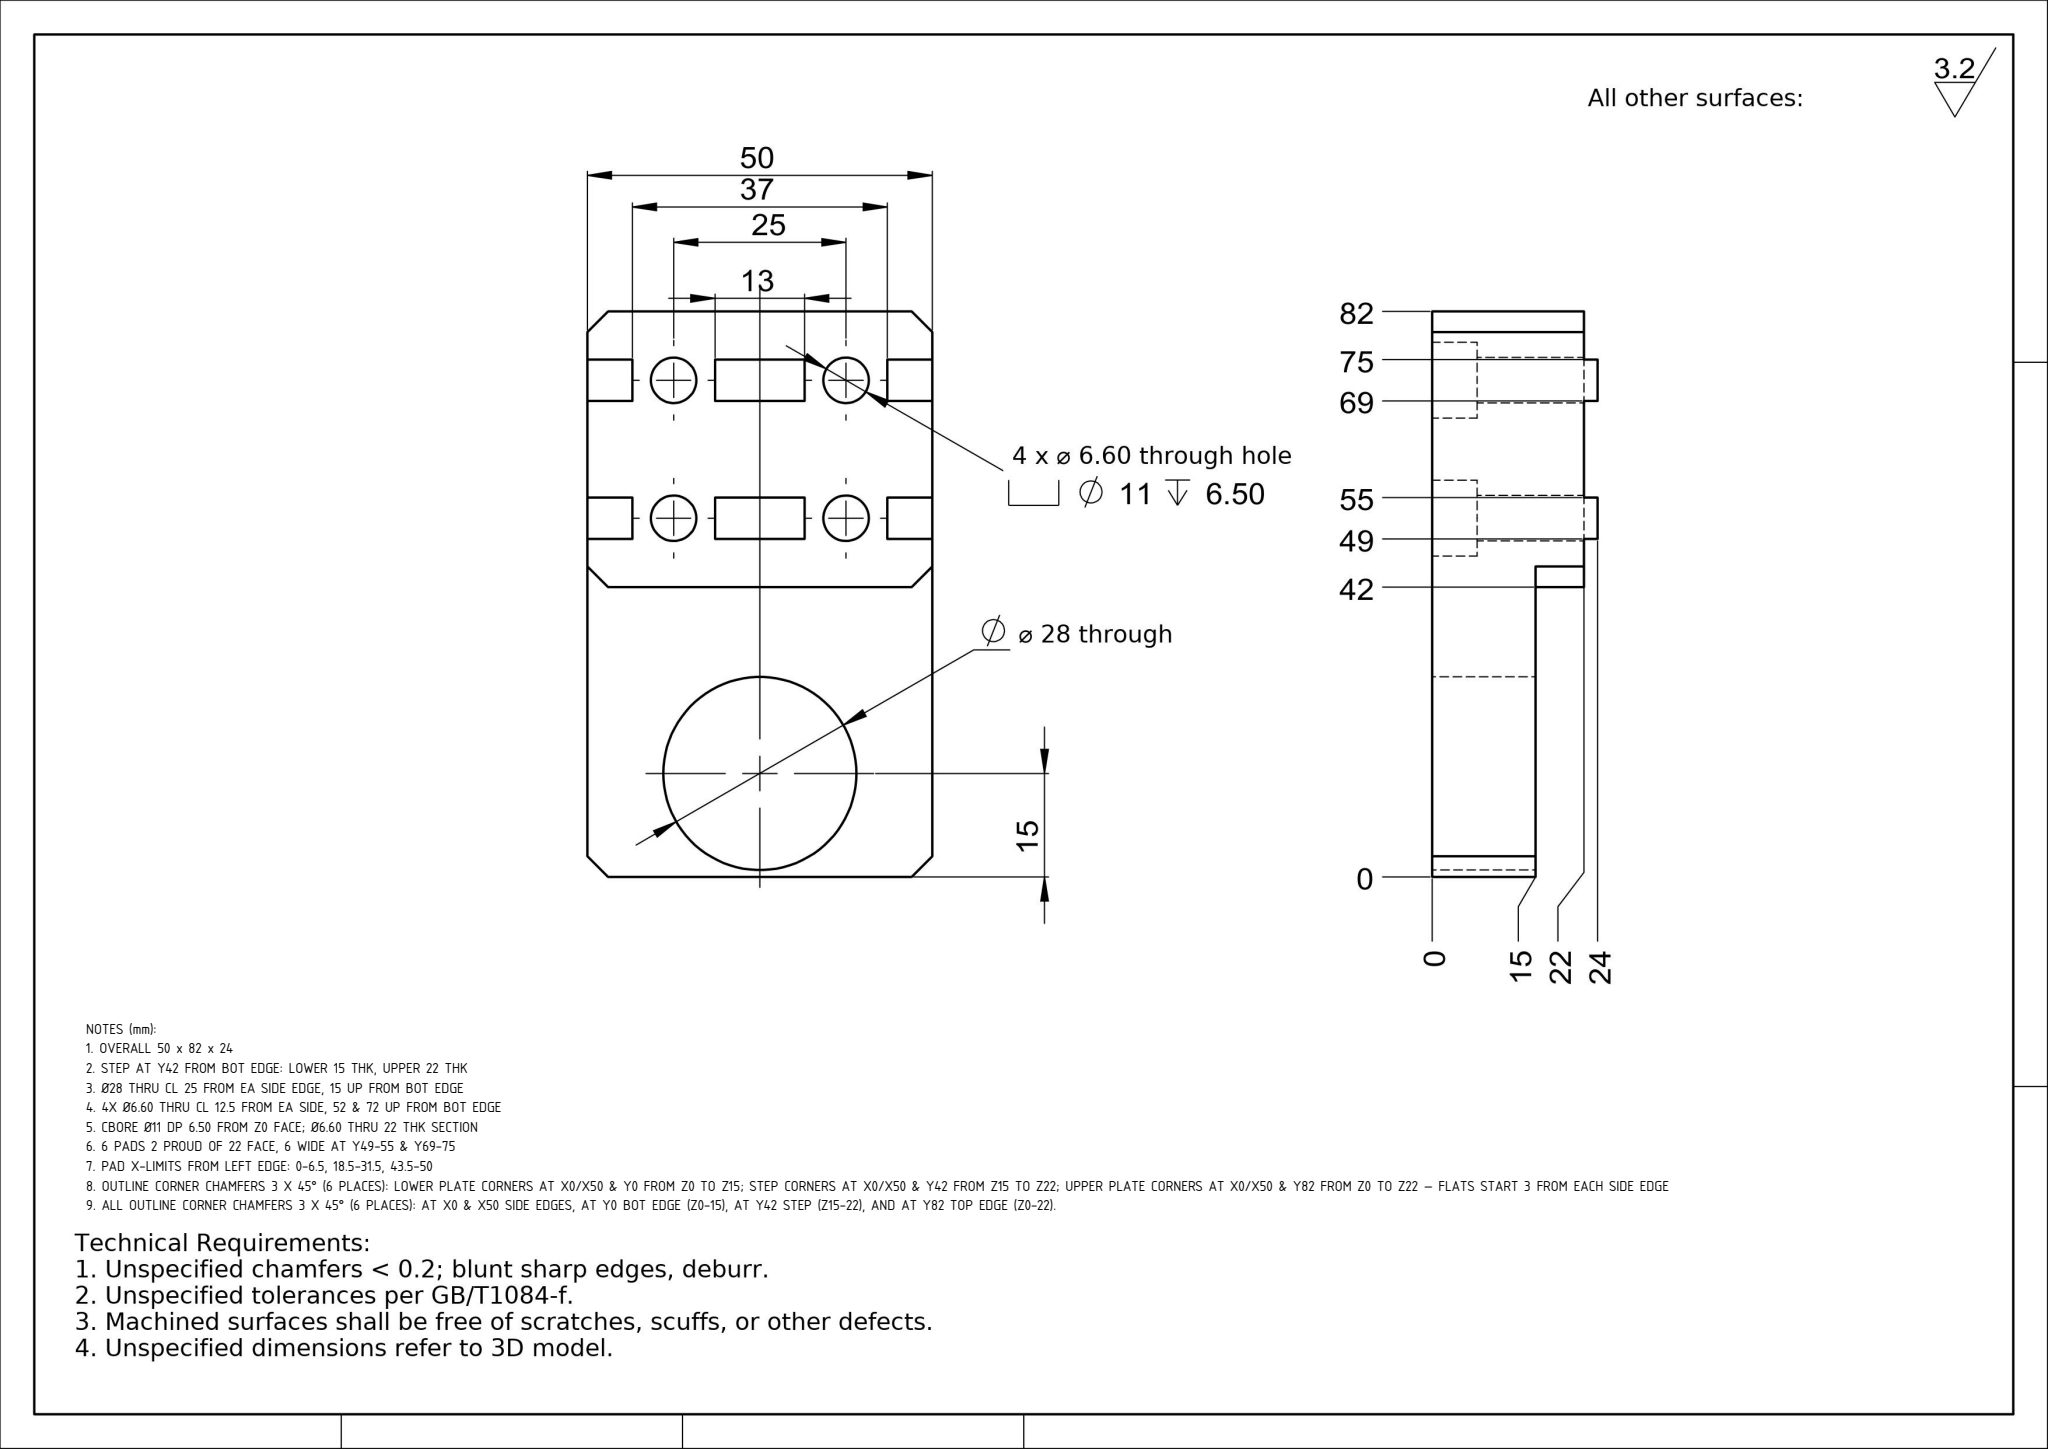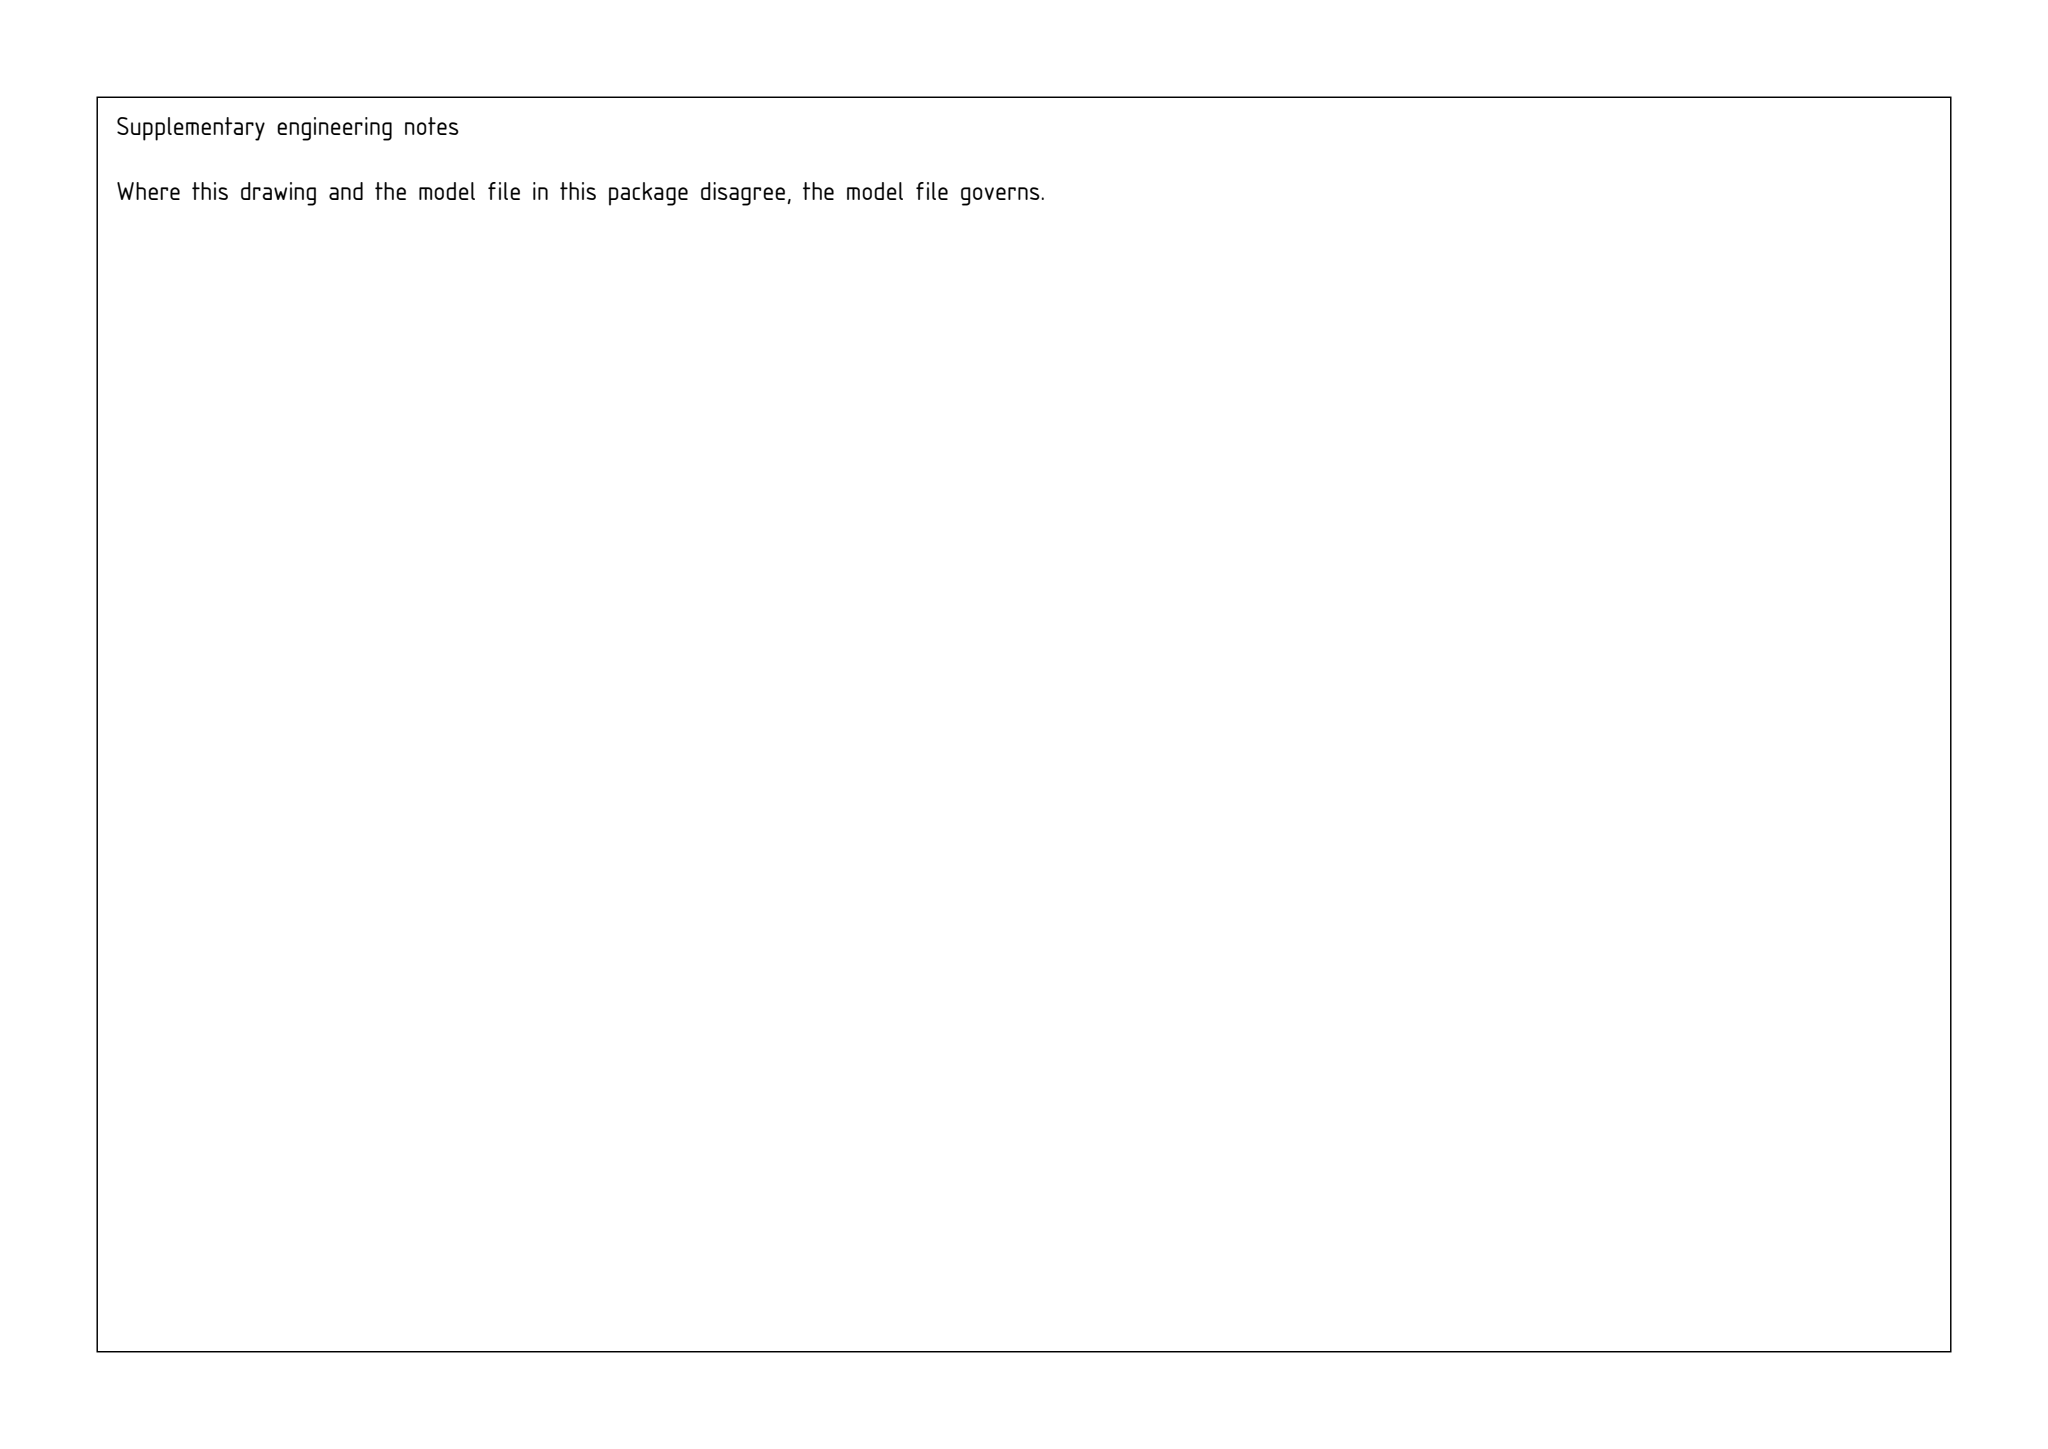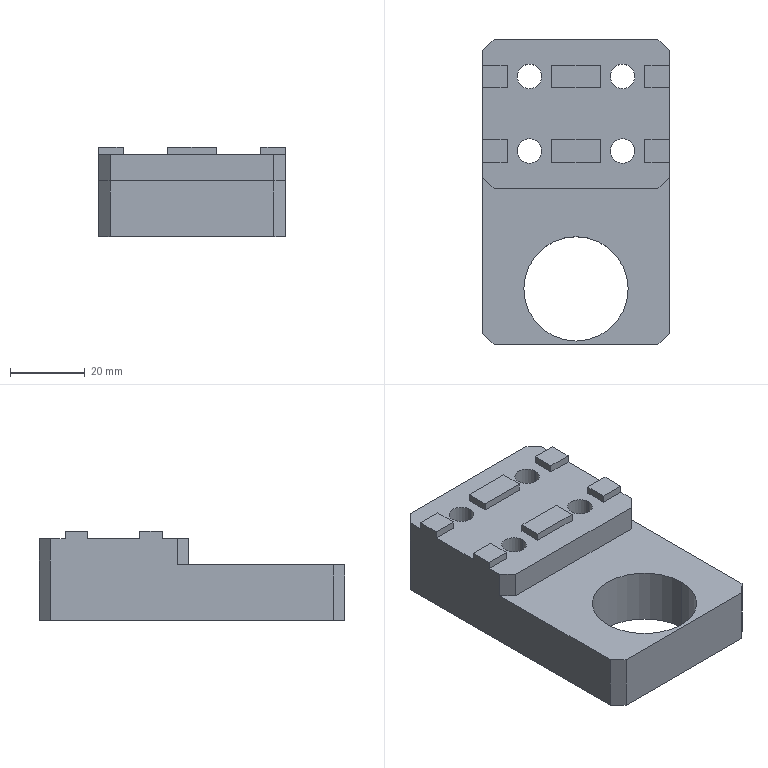Part | SolidWorks | mm | 1 solid | 62 faces | box 50 x 82 x 24 mm | volume 61900 mm3 | plane 44 | cylinder 18 | commonest cylinder face diameters 11 x8 6.6 x8 28 x2
Drawing notes:
OVERALL 50 x 82 x 24 | from the solid: bbox_xyz 50/82/24
STEP AT Y42 FROM BOT EDGE: LOWER 15 THK, UPPER 22 THK | from the solid: y plane 42.0; z planes 0/15/22
Ø28 THRU CL 25 FROM EA SIDE EDGE, 15 UP FROM BOT EDGE | from the solid: cyl Ø28 axis z at (25.0,15.0), len 15, bbox x=50
4X Ø6.60 THRU CL 12.5 FROM EA SIDE, 52 & 72 UP FROM BOT EDGE | from the solid: cyl Ø6.6 axis z at (12.5,52),(12.5,72),(37.5,52),(37.5,72); bbox 50x82
CBORE Ø11 DP 6.50 FROM Z0 FACE; Ø6.60 THRU 22 THK SECTION | from the solid: cyl Ø11 len 6.5 with z plane 6.5; Ø6.6 len 15.5 (6.5+15.5=22)
6 PADS 2 PROUD OF 22 FACE, 6 WIDE AT Y49-55 & Y69-75 | from the solid: z plane 22 (1 face) & 24 (6 faces); y planes 49/55/69/75
PAD X-LIMITS FROM LEFT EDGE: 0-6.5, 18.5-31.5, 43.5-50 | from the solid: x planes 0, 6.5, 18.5, 31.5, 43.5, 50
OUTLINE CORNER CHAMFERS 3 X 45° (6 PLACES): LOWER PLATE CORNERS AT X0/X50 & Y0 FROM Z0 TO Z15; STEP CORNERS AT X0/X50 & Y42 FROM Z15 TO Z22; UPPER PLATE CORNERS AT X0/X50 & Y82 FROM Z0 TO Z22 — FLATS START 3 FROM EACH SIDE EDGE | from the solid: inclined_planes: 6 faces at angle_to_xyz_axes [45,45,90], size 3x3 x (15 / 7 / 22), bbox_from [0,0,0],[47,0,0],[0,42,15],[47,42,15],[0,79,0],[47,79,0]
ALL OUTLINE CORNER CHAMFERS 3 X 45° (6 PLACES): AT X0 & X50 SIDE EDGES, AT Y0 BOT EDGE (Z0-15), AT Y42 STEP (Z15-22), AND AT Y82 TOP EDGE (Z0-22). | from the solid: inclined_planes: six 45/45/90 faces, size 3 x 3, bbox_from [0,0,0] & [47,0,0] (h15), [0,42,15] & [47,42,15] (h7), [0,79,0] & [47,79,0] (h22)
build123d program:
from build123d import *

# Parameters (mm, degrees)
SKETCH1_W                                       = 50
SKETCH1_H                                       = 82
BOSS_EXTRUDE1_DEPTH                             = 24
SKETCH2_W                                       = 50
SKETCH2_H                                       = 42
CUT_EXTRUDE1_DEPTH                              = 9
SKETCH3_R                                       = 14
CUT_EXTRUDE2_DEPTH                              = 54.684
M6_HEX_SOCKET_HEAD_CAP_SCREW_CBORE5_D           = 6.6
M6_HEX_SOCKET_HEAD_CAP_SCREW_CBORE5_CBORE_D     = 11
M6_HEX_SOCKET_HEAD_CAP_SCREW_CBORE5_CBORE_DEPTH = 6.5
SKETCH10_OUTSIDE_W                              = 71.798
SKETCH10_OUTSIDE_H                              = 103.798
SKETCH10_OUTSIDE_W_2                            = 50
SKETCH10_OUTSIDE_H_2                            = 6
CUT_EXTRUDE3_DEPTH                              = 2
CHAMFER1_SIZE                                   = 3
SKETCH11_W                                      = 12
SKETCH11_H                                      = 26
CUT_EXTRUDE4_DEPTH                              = 2


with BuildPart() as part:
    # Sketch1 → Boss-Extrude1 (new body)
    with BuildSketch(Plane.XY):
        Rectangle(SKETCH1_W, SKETCH1_H)
    extrude(amount=BOSS_EXTRUDE1_DEPTH)

    # Sketch2 → Cut-Extrude1 (cut)
    with BuildSketch(Plane.XY.offset(24)):
        with Locations((0, -20)):
            Rectangle(SKETCH2_W, SKETCH2_H)
    extrude(amount=-CUT_EXTRUDE1_DEPTH, mode=Mode.SUBTRACT)

    # Sketch3 → Cut-Extrude2 (cut, through all)
    with BuildSketch(Plane.XY.offset(24)):
        with Locations((0, -26)):
            Circle(SKETCH3_R)
    extrude(amount=-CUT_EXTRUDE2_DEPTH, mode=Mode.SUBTRACT)

    # M6 Hex Socket Head Cap Screw CBORE5 (through all)
    with Locations(Plane(origin=(0, 0, 0), x_dir=(-1, 0, 0), z_dir=(0, 0, -1))):
        with Locations((-12.5, 31), (-12.5, 11), (12.5, 31), (12.5, 11)):
            CounterBoreHole(M6_HEX_SOCKET_HEAD_CAP_SCREW_CBORE5_D / 2, M6_HEX_SOCKET_HEAD_CAP_SCREW_CBORE5_CBORE_D / 2, M6_HEX_SOCKET_HEAD_CAP_SCREW_CBORE5_CBORE_DEPTH)

    # Sketch10 outside → Cut-Extrude3 (cut)
    with BuildSketch(Plane.XY.offset(24)):
        Rectangle(SKETCH10_OUTSIDE_W, SKETCH10_OUTSIDE_H)
        with Locations((0, 31)):
            Rectangle(SKETCH10_OUTSIDE_W_2, SKETCH10_OUTSIDE_H_2, mode=Mode.SUBTRACT)
        with Locations((0, 11)):
            Rectangle(SKETCH10_OUTSIDE_W_2, SKETCH10_OUTSIDE_H_2, mode=Mode.SUBTRACT)
    extrude(amount=-CUT_EXTRUDE3_DEPTH, mode=Mode.SUBTRACT)

    # Chamfer1
    chamfer1_edges = [part.edges().sort_by_distance(p)[0] for p in [
        (25, -41, 7.5),
        (-25, -41, 7.5),
        (25, 1, 18.5),
        (-25, 1, 18.5),
        (-25, 41, 11),
        (25, 41, 11),
    ]]
    chamfer(chamfer1_edges, length=CHAMFER1_SIZE)

    # Sketch11 → Cut-Extrude4 (cut)
    with BuildSketch(Plane.XY.offset(24)):
        with Locations((-12.5, 21)):
            Rectangle(SKETCH11_W, SKETCH11_H)
        with Locations((12.5, 21)):
            Rectangle(SKETCH11_W, SKETCH11_H)
    extrude(amount=-CUT_EXTRUDE4_DEPTH, mode=Mode.SUBTRACT)


solid = part.part